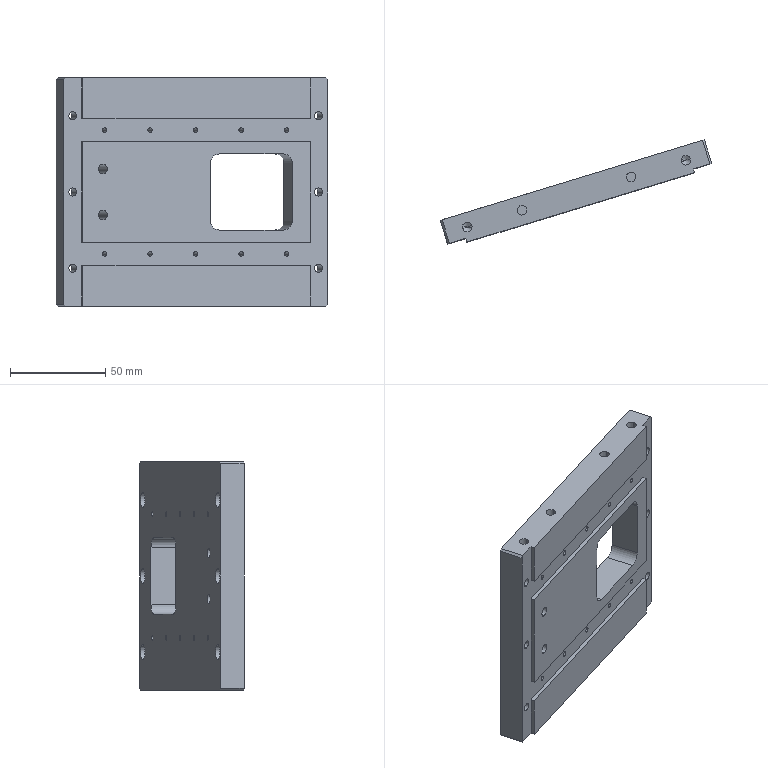Component | SolidWorks | V1ZHXTRotatingBasePlateSB1-1 | 1 solid | 99 faces | box 142.48 x 54.75 x 120 mm | volume 219079 mm3 | cylinder 60 | plane 35 | cone 4 | commonest cylinder face diameters 2.5 x20 7.8 x12 4.3 x12 5 x12 10 x4
build123d program:
from build123d import *

# Parameters (mm, degrees)
SKETCH1_W                                 = 145
SKETCH1_H                                 = 120
BOSS_EXTRUDE1_DEPTH                       = 15
M3_TAPPED_HOLE1_D                         = 2.5
LPATTERN1_COUNT                           = 5
LPATTERN1_PITCH                           = 25
SKETCH5_W                                 = 145
SKETCH5_H                                 = 12
CUT_EXTRUDE1_DEPTH                        = 2
SKETCH6_W                                 = 45
SKETCH6_H                                 = 40
CUT_EXTRUDE2_DEPTH                        = 96.296
FILLET1_R                                 = 5
M6_TAPPED_HOLE1_D                         = 5
SKETCH9_W                                 = 10
SKETCH9_H                                 = 120
CUT_EXTRUDE3_DEPTH                        = 2
M6_TAPPED_HOLE2_D                         = 5
M6_TAPPED_HOLE2_DEPTH                     = 13.5
M6_TAPPED_HOLE2_TIP                       = 1.502
SKETCH13_R                                = 2.5
CUT_EXTRUDE4_DEPTH                        = 15
HOLE_SIZE_FOR_HEX_SOCKET_HEAD_CAP_2_COUNT = 2
HOLE_SIZE_FOR_HEX_SOCKET_HEAD_CAP_2_PITCH = 40
HOLE_SIZE_FOR_HEX_SOCKET_HEAD_CAP_3_COUNT = 2
HOLE_SIZE_FOR_HEX_SOCKET_HEAD_CAP_3_PITCH = 80
CHAMFER1_SIZE                             = 1


with BuildPart() as part:
    # Sketch1 → Boss-Extrude1 (new body)
    with BuildSketch(Plane(origin=(0, 0, 0), x_dir=(1, 0, 0), z_dir=(0, 1, 0))):
        Rectangle(SKETCH1_W, SKETCH1_H)
    extrude(amount=BOSS_EXTRUDE1_DEPTH)

    # M3 Tapped Hole1 (through all)
    with Locations(Plane(origin=(0, 15, 0), x_dir=(1, 0, 0), z_dir=(0, 1, 0))):
        with Locations((-50, -32.5), (-50, 32.5)):
            m3_tapped_hole1 = Hole(M3_TAPPED_HOLE1_D / 2)

    # LPattern1: M3 Tapped Hole1 ×5
    with Locations(*[(i * LPATTERN1_PITCH, 0, 0) for i in range(1, LPATTERN1_COUNT)]):
        add(m3_tapped_hole1, mode=Mode.SUBTRACT)

    # Sketch5 → Cut-Extrude1 (cut)
    with BuildSketch(Plane.XZ):
        with Locations((0, -32.5)):
            Rectangle(SKETCH5_W, SKETCH5_H)
    cut_extrude1 = extrude(amount=-CUT_EXTRUDE1_DEPTH, mode=Mode.SUBTRACT)

    # Mirror1: Cut-Extrude1 across plane
    add(cut_extrude1.mirror(Plane.XY), mode=Mode.SUBTRACT)

    # Sketch6 → Cut-Extrude2 (cut, through all)
    with BuildSketch(Plane(origin=(0, 15, 0), x_dir=(1, 0, 0), z_dir=(0, 1, 0))):
        with Locations((-30, 0)):
            Rectangle(SKETCH6_W, SKETCH6_H)
    extrude(amount=-CUT_EXTRUDE2_DEPTH, mode=Mode.SUBTRACT)

    # Fillet1
    fillet1_edges = [part.edges().sort_by_distance(p)[0] for p in [
        (-7.5, 7.5, -20),
        (-7.5, 7.5, 20),
        (-52.5, 7.5, 20),
        (-52.5, 7.5, -20),
    ]]
    fillet(fillet1_edges, radius=FILLET1_R)

    # M6 Tapped Hole1 (through all)
    with Locations(Plane(origin=(0, 15, 0), x_dir=(1, 0, 0), z_dir=(0, 1, 0))):
        with Locations((51.5, 12), (51.5, -12)):
            Hole(M6_TAPPED_HOLE1_D / 2)

    # Sketch9 → Cut-Extrude3 (cut)
    with BuildSketch(Plane.XZ):
        with Locations((-67.5, 0)):
            Rectangle(SKETCH9_W, SKETCH9_H)
        with Locations((67.5, 0)):
            Rectangle(SKETCH9_W, SKETCH9_H)
    extrude(amount=-CUT_EXTRUDE3_DEPTH, mode=Mode.SUBTRACT)

    # M6 Tapped Hole2
    with Locations(Plane(origin=(0, 0, -60), x_dir=(-1, 0, 0), z_dir=(0, 0, -1))):
        with Locations((60, 7.5), (-60, 7.5)):
            Hole(M6_TAPPED_HOLE2_D / 2, depth=M6_TAPPED_HOLE2_DEPTH)
            with Locations((0, 0, -(M6_TAPPED_HOLE2_DEPTH + M6_TAPPED_HOLE2_TIP / 2))):  # 118° drill point
                Cone(0, M6_TAPPED_HOLE2_D / 2, M6_TAPPED_HOLE2_TIP, mode=Mode.SUBTRACT)

    # Sketch13 → Cut-Extrude4 (cut)
    with BuildSketch(Plane(origin=(0, 0, -60), x_dir=(-1, 0, 0), z_dir=(0, 0, -1))):
        with Locations((-30, 7.5)):
            Circle(SKETCH13_R)
        with Locations((30, 7.5)):
            Circle(SKETCH13_R)
    extrude(amount=-CUT_EXTRUDE4_DEPTH, mode=Mode.SUBTRACT)

    # Sketch14 → Hole Size _for_ Hex Socket Head Cap Scre (revolve, cut)
    with BuildSketch(Plane(origin=(-67.5, 15, -40), x_dir=(0, 0, 1), z_dir=(1, 0, 0))):
        Polygon((0, 0), (0, 19.292), (2.15, 18), (2.15, 4.6), (3.9, 4.6), (3.9, 0), align=None)
    hole_size_for_hex_socket_head_cap_scre = revolve(axis=Axis((-67.5, 21.35, -40), (0, -1, 0)), mode=Mode.SUBTRACT)

    # Hole Size _for_ Hex Socket Head Cap  2: Hole Size _for_ Hex Socket Head Cap Scre ×2
    with Locations(*[(0, 0, i * HOLE_SIZE_FOR_HEX_SOCKET_HEAD_CAP_2_PITCH) for i in range(1, HOLE_SIZE_FOR_HEX_SOCKET_HEAD_CAP_2_COUNT)]):
        add(hole_size_for_hex_socket_head_cap_scre, mode=Mode.SUBTRACT)

    # Hole Size _for_ Hex Socket Head Cap  3: Hole Size _for_ Hex Socket Head Cap Scre ×2
    with Locations(*[(0, 0, i * HOLE_SIZE_FOR_HEX_SOCKET_HEAD_CAP_3_PITCH) for i in range(1, HOLE_SIZE_FOR_HEX_SOCKET_HEAD_CAP_3_COUNT)]):
        add(hole_size_for_hex_socket_head_cap_scre, mode=Mode.SUBTRACT)

    # Mirror2: Hole Size _for_ Hex Socket Head Cap Scre across plane
    add(hole_size_for_hex_socket_head_cap_scre.mirror(Plane(origin=(0, 0, 0), x_dir=(0, 0, 1), z_dir=(1, 0, 0))), mode=Mode.SUBTRACT)

    # Mirror2 copy 1 sketch → Mirror2 copy 1 (revolve, cut)
    with BuildSketch(Plane(origin=(67.5, 15, 0), x_dir=(0, 0, 1), z_dir=(-1, 0, 0))):
        Polygon((0, 0), (0, -19.292), (2.15, -18), (2.15, -4.6), (3.9, -4.6), (3.9, 0), align=None)
    revolve(axis=Axis((67.5, 21.35, 0), (0, 1, 0)), mode=Mode.SUBTRACT)

    # Mirror2 copy 2 sketch → Mirror2 copy 2 (revolve, cut)
    with BuildSketch(Plane(origin=(67.5, 15, 40), x_dir=(0, 0, 1), z_dir=(-1, 0, 0))):
        Polygon((0, 0), (0, -19.292), (2.15, -18), (2.15, -4.6), (3.9, -4.6), (3.9, 0), align=None)
    revolve(axis=Axis((67.5, 21.35, 40), (0, 1, 0)), mode=Mode.SUBTRACT)

    # Chamfer1
    chamfer1_edges = [part.edges().sort_by_distance(p)[0] for p in [
        (72.5, 8.5, 60),
        (-72.5, 8.5, 60),
        (-72.5, 8.5, -60),
        (72.5, 8.5, -60),
    ]]
    chamfer(chamfer1_edges, length=CHAMFER1_SIZE)


solid = part.part

# Placed as in the assembly
solid = solid.moved(Location((165.14, -166.829, 375.239), (-180, 0, 163.032)))